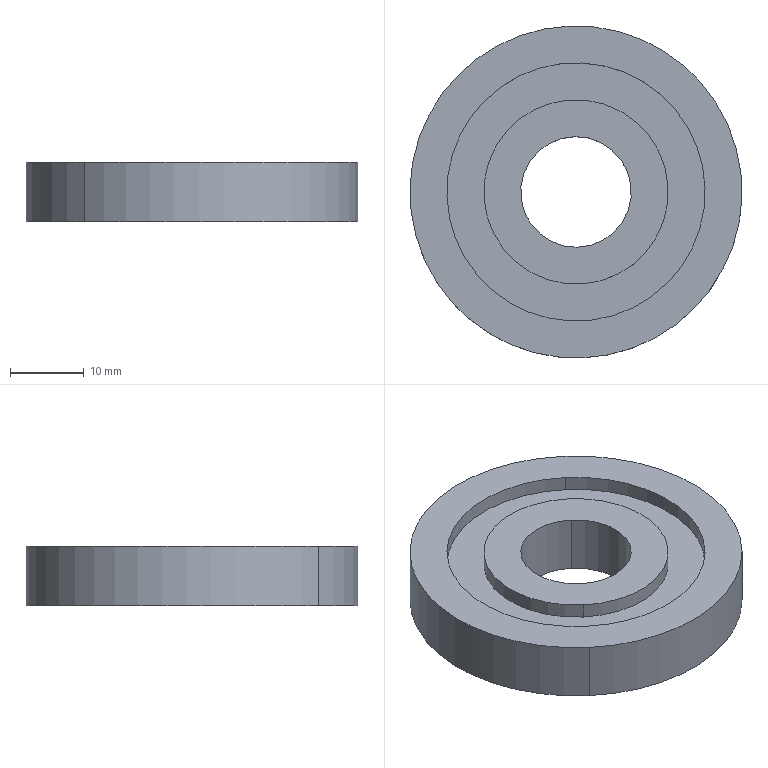Component | SolidWorks | ExcessDoughCuttingWheelBearing-3 | 1 solid | 18 faces | box 45 x 45 x 8 mm | volume 9425 mm3 | cylinder 12 | plane 6 | commonest cylinder face diameters 25 x4 35 x4 15 x2 45 x2
STEP:
#1=CARTESIAN_POINT('',(9.886,-13.898,62.312));
#2=VERTEX_POINT('',#1);
#3=CARTESIAN_POINT('',(9.503,-14.347,62.312));
#4=VERTEX_POINT('',#3);
#5=CARTESIAN_POINT('',(9.695,-14.123,62.312));
#6=DIRECTION('',(0.,0.,1.));
#7=DIRECTION('',(-0.6489,-0.7608,0.));
#8=AXIS2_PLACEMENT_3D('',#5,#6,#7);
#9=CIRCLE('',#8,0.2953);
#10=EDGE_CURVE('',#2,#4,#9,.T.);
#11=ORIENTED_EDGE('',*,*,#10,.F.);
#12=CARTESIAN_POINT('',(9.886,-13.898,62.627));
#13=VERTEX_POINT('',#12);
#14=CARTESIAN_POINT('',(9.886,-13.898,62.684));
#15=DIRECTION('',(0.,0.,1.));
#16=VECTOR('',#15,39.37);
#17=LINE('',#14,#16);
#18=EDGE_CURVE('',#2,#13,#17,.T.);
#19=ORIENTED_EDGE('',*,*,#18,.T.);
#20=CARTESIAN_POINT('',(9.503,-14.347,62.627));
#21=VERTEX_POINT('',#20);
#22=CARTESIAN_POINT('',(9.695,-14.123,62.627));
#23=DIRECTION('',(0.,0.,1.));
#24=DIRECTION('',(-0.6489,-0.7608,0.));
#25=AXIS2_PLACEMENT_3D('',#22,#23,#24);
#26=CIRCLE('',#25,0.2953);
#27=EDGE_CURVE('',#13,#21,#26,.T.);
#28=ORIENTED_EDGE('',*,*,#27,.T.);
#29=CARTESIAN_POINT('',(9.503,-14.347,62.684));
#30=DIRECTION('',(0.,0.,1.));
#31=VECTOR('',#30,39.37);
#32=LINE('',#29,#31);
#33=EDGE_CURVE('',#4,#21,#32,.T.);
#34=ORIENTED_EDGE('',*,*,#33,.F.);
#35=EDGE_LOOP('',(#11,#19,#28,#34));
#36=FACE_OUTER_BOUND('',#35,.T.);
#37=CARTESIAN_POINT('',(9.695,-14.123,62.684));
#38=DIRECTION('',(0.,0.,1.));
#39=DIRECTION('',(-0.6489,-0.7608,0.));
#40=AXIS2_PLACEMENT_3D('',#37,#38,#39);
#41=CYLINDRICAL_SURFACE('',#40,0.2953);
#42=ADVANCED_FACE('',(#36),#41,.F.);
#43=CARTESIAN_POINT('',(9.375,-14.497,62.312));
#44=VERTEX_POINT('',#43);
#45=CARTESIAN_POINT('',(10.014,-13.748,62.312));
#46=VERTEX_POINT('',#45);
#47=CARTESIAN_POINT('',(9.695,-14.123,62.312));
#48=DIRECTION('',(0.,0.,1.));
#49=DIRECTION('',(-0.6489,-0.7608,0.));
#50=AXIS2_PLACEMENT_3D('',#47,#48,#49);
#51=CIRCLE('',#50,0.4921);
#52=EDGE_CURVE('',#44,#46,#51,.T.);
#53=ORIENTED_EDGE('',*,*,#52,.T.);
#54=CARTESIAN_POINT('',(10.014,-13.748,62.391));
#55=VERTEX_POINT('',#54);
#56=CARTESIAN_POINT('',(10.014,-13.748,62.684));
#57=DIRECTION('',(0.,0.,1.));
#58=VECTOR('',#57,39.37);
#59=LINE('',#56,#58);
#60=EDGE_CURVE('',#46,#55,#59,.T.);
#61=ORIENTED_EDGE('',*,*,#60,.T.);
#62=CARTESIAN_POINT('',(9.375,-14.497,62.391));
#63=VERTEX_POINT('',#62);
#64=CARTESIAN_POINT('',(9.695,-14.123,62.391));
#65=DIRECTION('',(0.,0.,1.));
#66=DIRECTION('',(-0.6489,-0.7608,0.));
#67=AXIS2_PLACEMENT_3D('',#64,#65,#66);
#68=CIRCLE('',#67,0.4921);
#69=EDGE_CURVE('',#63,#55,#68,.T.);
#70=ORIENTED_EDGE('',*,*,#69,.F.);
#71=CARTESIAN_POINT('',(9.375,-14.497,62.684));
#72=DIRECTION('',(0.,0.,1.));
#73=VECTOR('',#72,39.37);
#74=LINE('',#71,#73);
#75=EDGE_CURVE('',#44,#63,#74,.T.);
#76=ORIENTED_EDGE('',*,*,#75,.F.);
#77=EDGE_LOOP('',(#53,#61,#70,#76));
#78=FACE_OUTER_BOUND('',#77,.T.);
#79=CARTESIAN_POINT('',(9.695,-14.123,62.684));
#80=DIRECTION('',(0.,0.,1.));
#81=DIRECTION('',(-0.6489,-0.7608,0.));
#82=AXIS2_PLACEMENT_3D('',#79,#80,#81);
#83=CYLINDRICAL_SURFACE('',#82,0.4921);
#84=ADVANCED_FACE('',(#78),#83,.T.);
#85=CARTESIAN_POINT('',(10.142,-13.598,62.312));
#86=VERTEX_POINT('',#85);
#87=CARTESIAN_POINT('',(9.247,-14.647,62.312));
#88=VERTEX_POINT('',#87);
#89=CARTESIAN_POINT('',(9.695,-14.123,62.312));
#90=DIRECTION('',(0.,0.,1.));
#91=DIRECTION('',(-0.6489,-0.7608,0.));
#92=AXIS2_PLACEMENT_3D('',#89,#90,#91);
#93=CIRCLE('',#92,0.689);
#94=EDGE_CURVE('',#86,#88,#93,.T.);
#95=ORIENTED_EDGE('',*,*,#94,.F.);
#96=CARTESIAN_POINT('',(10.142,-13.598,62.391));
#97=VERTEX_POINT('',#96);
#98=CARTESIAN_POINT('',(10.142,-13.598,62.684));
#99=DIRECTION('',(0.,0.,1.));
#100=VECTOR('',#99,39.37);
#101=LINE('',#98,#100);
#102=EDGE_CURVE('',#86,#97,#101,.T.);
#103=ORIENTED_EDGE('',*,*,#102,.T.);
#104=CARTESIAN_POINT('',(9.247,-14.647,62.391));
#105=VERTEX_POINT('',#104);
#106=CARTESIAN_POINT('',(9.695,-14.123,62.391));
#107=DIRECTION('',(0.,0.,1.));
#108=DIRECTION('',(-0.6489,-0.7608,0.));
#109=AXIS2_PLACEMENT_3D('',#106,#107,#108);
#110=CIRCLE('',#109,0.689);
#111=EDGE_CURVE('',#97,#105,#110,.T.);
#112=ORIENTED_EDGE('',*,*,#111,.T.);
#113=CARTESIAN_POINT('',(9.247,-14.647,62.684));
#114=DIRECTION('',(0.,0.,1.));
#115=VECTOR('',#114,39.37);
#116=LINE('',#113,#115);
#117=EDGE_CURVE('',#88,#105,#116,.T.);
#118=ORIENTED_EDGE('',*,*,#117,.F.);
#119=EDGE_LOOP('',(#95,#103,#112,#118));
#120=FACE_OUTER_BOUND('',#119,.T.);
#121=CARTESIAN_POINT('',(9.695,-14.123,62.684));
#122=DIRECTION('',(0.,0.,1.));
#123=DIRECTION('',(-0.6489,-0.7608,0.));
#124=AXIS2_PLACEMENT_3D('',#121,#122,#123);
#125=CYLINDRICAL_SURFACE('',#124,0.689);
#126=ADVANCED_FACE('',(#120),#125,.F.);
#127=CARTESIAN_POINT('',(9.12,-14.797,62.312));
#128=VERTEX_POINT('',#127);
#129=CARTESIAN_POINT('',(10.269,-13.449,62.312));
#130=VERTEX_POINT('',#129);
#131=CARTESIAN_POINT('',(9.695,-14.123,62.312));
#132=DIRECTION('',(0.,0.,1.));
#133=DIRECTION('',(-0.6489,-0.7608,0.));
#134=AXIS2_PLACEMENT_3D('',#131,#132,#133);
#135=CIRCLE('',#134,0.8858);
#136=EDGE_CURVE('',#128,#130,#135,.T.);
#137=ORIENTED_EDGE('',*,*,#136,.T.);
#138=CARTESIAN_POINT('',(10.269,-13.449,62.627));
#139=VERTEX_POINT('',#138);
#140=CARTESIAN_POINT('',(10.269,-13.449,62.684));
#141=DIRECTION('',(0.,0.,1.));
#142=VECTOR('',#141,39.37);
#143=LINE('',#140,#142);
#144=EDGE_CURVE('',#130,#139,#143,.T.);
#145=ORIENTED_EDGE('',*,*,#144,.T.);
#146=CARTESIAN_POINT('',(9.12,-14.797,62.627));
#147=VERTEX_POINT('',#146);
#148=CARTESIAN_POINT('',(9.695,-14.123,62.627));
#149=DIRECTION('',(0.,0.,1.));
#150=DIRECTION('',(-0.6489,-0.7608,0.));
#151=AXIS2_PLACEMENT_3D('',#148,#149,#150);
#152=CIRCLE('',#151,0.8858);
#153=EDGE_CURVE('',#147,#139,#152,.T.);
#154=ORIENTED_EDGE('',*,*,#153,.F.);
#155=CARTESIAN_POINT('',(9.12,-14.797,62.684));
#156=DIRECTION('',(0.,0.,1.));
#157=VECTOR('',#156,39.37);
#158=LINE('',#155,#157);
#159=EDGE_CURVE('',#128,#147,#158,.T.);
#160=ORIENTED_EDGE('',*,*,#159,.F.);
#161=EDGE_LOOP('',(#137,#145,#154,#160));
#162=FACE_OUTER_BOUND('',#161,.T.);
#163=CARTESIAN_POINT('',(9.695,-14.123,62.684));
#164=DIRECTION('',(0.,0.,1.));
#165=DIRECTION('',(-0.6489,-0.7608,0.));
#166=AXIS2_PLACEMENT_3D('',#163,#164,#165);
#167=CYLINDRICAL_SURFACE('',#166,0.8858);
#168=ADVANCED_FACE('',(#162),#167,.T.);
#169=CARTESIAN_POINT('',(10.142,-13.598,62.548));
#170=VERTEX_POINT('',#169);
#171=CARTESIAN_POINT('',(9.247,-14.647,62.548));
#172=VERTEX_POINT('',#171);
#173=CARTESIAN_POINT('',(9.695,-14.123,62.548));
#174=DIRECTION('',(0.,0.,1.));
#175=DIRECTION('',(-0.6489,-0.7608,0.));
#176=AXIS2_PLACEMENT_3D('',#173,#174,#175);
#177=CIRCLE('',#176,0.689);
#178=EDGE_CURVE('',#170,#172,#177,.T.);
#179=ORIENTED_EDGE('',*,*,#178,.F.);
#180=CARTESIAN_POINT('',(10.142,-13.598,62.627));
#181=VERTEX_POINT('',#180);
#182=CARTESIAN_POINT('',(10.142,-13.598,62.684));
#183=DIRECTION('',(0.,0.,1.));
#184=VECTOR('',#183,39.37);
#185=LINE('',#182,#184);
#186=EDGE_CURVE('',#170,#181,#185,.T.);
#187=ORIENTED_EDGE('',*,*,#186,.T.);
#188=CARTESIAN_POINT('',(9.247,-14.647,62.627));
#189=VERTEX_POINT('',#188);
#190=CARTESIAN_POINT('',(9.695,-14.123,62.627));
#191=DIRECTION('',(0.,0.,1.));
#192=DIRECTION('',(-0.6489,-0.7608,0.));
#193=AXIS2_PLACEMENT_3D('',#190,#191,#192);
#194=CIRCLE('',#193,0.689);
#195=EDGE_CURVE('',#181,#189,#194,.T.);
#196=ORIENTED_EDGE('',*,*,#195,.T.);
#197=CARTESIAN_POINT('',(9.247,-14.647,62.684));
#198=DIRECTION('',(0.,0.,1.));
#199=VECTOR('',#198,39.37);
#200=LINE('',#197,#199);
#201=EDGE_CURVE('',#172,#189,#200,.T.);
#202=ORIENTED_EDGE('',*,*,#201,.F.);
#203=EDGE_LOOP('',(#179,#187,#196,#202));
#204=FACE_OUTER_BOUND('',#203,.T.);
#205=CARTESIAN_POINT('',(9.695,-14.123,62.684));
#206=DIRECTION('',(0.,0.,1.));
#207=DIRECTION('',(-0.6489,-0.7608,0.));
#208=AXIS2_PLACEMENT_3D('',#205,#206,#207);
#209=CYLINDRICAL_SURFACE('',#208,0.689);
#210=ADVANCED_FACE('',(#204),#209,.F.);
#211=CARTESIAN_POINT('',(9.375,-14.497,62.548));
#212=VERTEX_POINT('',#211);
#213=CARTESIAN_POINT('',(10.014,-13.748,62.548));
#214=VERTEX_POINT('',#213);
#215=CARTESIAN_POINT('',(9.695,-14.123,62.548));
#216=DIRECTION('',(0.,0.,1.));
#217=DIRECTION('',(-0.6489,-0.7608,0.));
#218=AXIS2_PLACEMENT_3D('',#215,#216,#217);
#219=CIRCLE('',#218,0.4921);
#220=EDGE_CURVE('',#212,#214,#219,.T.);
#221=ORIENTED_EDGE('',*,*,#220,.T.);
#222=CARTESIAN_POINT('',(10.014,-13.748,62.627));
#223=VERTEX_POINT('',#222);
#224=CARTESIAN_POINT('',(10.014,-13.748,62.684));
#225=DIRECTION('',(0.,0.,1.));
#226=VECTOR('',#225,39.37);
#227=LINE('',#224,#226);
#228=EDGE_CURVE('',#214,#223,#227,.T.);
#229=ORIENTED_EDGE('',*,*,#228,.T.);
#230=CARTESIAN_POINT('',(9.375,-14.497,62.627));
#231=VERTEX_POINT('',#230);
#232=CARTESIAN_POINT('',(9.695,-14.123,62.627));
#233=DIRECTION('',(0.,0.,1.));
#234=DIRECTION('',(-0.6489,-0.7608,0.));
#235=AXIS2_PLACEMENT_3D('',#232,#233,#234);
#236=CIRCLE('',#235,0.4921);
#237=EDGE_CURVE('',#231,#223,#236,.T.);
#238=ORIENTED_EDGE('',*,*,#237,.F.);
#239=CARTESIAN_POINT('',(9.375,-14.497,62.684));
#240=DIRECTION('',(0.,0.,1.));
#241=VECTOR('',#240,39.37);
#242=LINE('',#239,#241);
#243=EDGE_CURVE('',#212,#231,#242,.T.);
#244=ORIENTED_EDGE('',*,*,#243,.F.);
#245=EDGE_LOOP('',(#221,#229,#238,#244));
#246=FACE_OUTER_BOUND('',#245,.T.);
#247=CARTESIAN_POINT('',(9.695,-14.123,62.684));
#248=DIRECTION('',(0.,0.,1.));
#249=DIRECTION('',(-0.6489,-0.7608,0.));
#250=AXIS2_PLACEMENT_3D('',#247,#248,#249);
#251=CYLINDRICAL_SURFACE('',#250,0.4921);
#252=ADVANCED_FACE('',(#246),#251,.T.);
#253=CARTESIAN_POINT('',(9.695,-14.123,62.627));
#254=DIRECTION('',(0.,0.,1.));
#255=DIRECTION('',(-0.6489,-0.7608,0.));
#256=AXIS2_PLACEMENT_3D('',#253,#254,#255);
#257=CIRCLE('',#256,0.2953);
#258=EDGE_CURVE('',#21,#13,#257,.T.);
#259=ORIENTED_EDGE('',*,*,#258,.F.);
#260=ORIENTED_EDGE('',*,*,#27,.F.);
#261=EDGE_LOOP('',(#259,#260));
#262=FACE_BOUND('',#261,.T.);
#263=ORIENTED_EDGE('',*,*,#237,.T.);
#264=CARTESIAN_POINT('',(9.695,-14.123,62.627));
#265=DIRECTION('',(0.,0.,1.));
#266=DIRECTION('',(-0.6489,-0.7608,0.));
#267=AXIS2_PLACEMENT_3D('',#264,#265,#266);
#268=CIRCLE('',#267,0.4921);
#269=EDGE_CURVE('',#223,#231,#268,.T.);
#270=ORIENTED_EDGE('',*,*,#269,.T.);
#271=EDGE_LOOP('',(#263,#270));
#272=FACE_OUTER_BOUND('',#271,.T.);
#273=CARTESIAN_POINT('',(9.886,-13.898,62.627));
#274=DIRECTION('',(0.,0.,-1.));
#275=DIRECTION('',(0.6489,0.7608,0.));
#276=AXIS2_PLACEMENT_3D('',#273,#274,#275);
#277=PLANE('',#276);
#278=ADVANCED_FACE('',(#262,#272),#277,.F.);
#279=ORIENTED_EDGE('',*,*,#228,.F.);
#280=CARTESIAN_POINT('',(9.695,-14.123,62.548));
#281=DIRECTION('',(0.,0.,1.));
#282=DIRECTION('',(-0.6489,-0.7608,0.));
#283=AXIS2_PLACEMENT_3D('',#280,#281,#282);
#284=CIRCLE('',#283,0.4921);
#285=EDGE_CURVE('',#214,#212,#284,.T.);
#286=ORIENTED_EDGE('',*,*,#285,.T.);
#287=ORIENTED_EDGE('',*,*,#243,.T.);
#288=ORIENTED_EDGE('',*,*,#269,.F.);
#289=EDGE_LOOP('',(#279,#286,#287,#288));
#290=FACE_OUTER_BOUND('',#289,.T.);
#291=CARTESIAN_POINT('',(9.695,-14.123,62.684));
#292=DIRECTION('',(0.,0.,1.));
#293=DIRECTION('',(-0.6489,-0.7608,0.));
#294=AXIS2_PLACEMENT_3D('',#291,#292,#293);
#295=CYLINDRICAL_SURFACE('',#294,0.4921);
#296=ADVANCED_FACE('',(#290),#295,.T.);
#297=ORIENTED_EDGE('',*,*,#220,.F.);
#298=ORIENTED_EDGE('',*,*,#285,.F.);
#299=EDGE_LOOP('',(#297,#298));
#300=FACE_BOUND('',#299,.T.);
#301=CARTESIAN_POINT('',(9.695,-14.123,62.548));
#302=DIRECTION('',(0.,0.,1.));
#303=DIRECTION('',(-0.6489,-0.7608,0.));
#304=AXIS2_PLACEMENT_3D('',#301,#302,#303);
#305=CIRCLE('',#304,0.689);
#306=EDGE_CURVE('',#172,#170,#305,.T.);
#307=ORIENTED_EDGE('',*,*,#306,.T.);
#308=ORIENTED_EDGE('',*,*,#178,.T.);
#309=EDGE_LOOP('',(#307,#308));
#310=FACE_OUTER_BOUND('',#309,.T.);
#311=CARTESIAN_POINT('',(10.014,-13.748,62.548));
#312=DIRECTION('',(0.,0.,-1.));
#313=DIRECTION('',(0.6489,0.7608,0.));
#314=AXIS2_PLACEMENT_3D('',#311,#312,#313);
#315=PLANE('',#314);
#316=ADVANCED_FACE('',(#300,#310),#315,.F.);
#317=ORIENTED_EDGE('',*,*,#186,.F.);
#318=ORIENTED_EDGE('',*,*,#306,.F.);
#319=ORIENTED_EDGE('',*,*,#201,.T.);
#320=CARTESIAN_POINT('',(9.695,-14.123,62.627));
#321=DIRECTION('',(0.,0.,1.));
#322=DIRECTION('',(-0.6489,-0.7608,0.));
#323=AXIS2_PLACEMENT_3D('',#320,#321,#322);
#324=CIRCLE('',#323,0.689);
#325=EDGE_CURVE('',#189,#181,#324,.T.);
#326=ORIENTED_EDGE('',*,*,#325,.T.);
#327=EDGE_LOOP('',(#317,#318,#319,#326));
#328=FACE_OUTER_BOUND('',#327,.T.);
#329=CARTESIAN_POINT('',(9.695,-14.123,62.684));
#330=DIRECTION('',(0.,0.,1.));
#331=DIRECTION('',(-0.6489,-0.7608,0.));
#332=AXIS2_PLACEMENT_3D('',#329,#330,#331);
#333=CYLINDRICAL_SURFACE('',#332,0.689);
#334=ADVANCED_FACE('',(#328),#333,.F.);
#335=ORIENTED_EDGE('',*,*,#325,.F.);
#336=ORIENTED_EDGE('',*,*,#195,.F.);
#337=EDGE_LOOP('',(#335,#336));
#338=FACE_BOUND('',#337,.T.);
#339=ORIENTED_EDGE('',*,*,#153,.T.);
#340=CARTESIAN_POINT('',(9.695,-14.123,62.627));
#341=DIRECTION('',(0.,0.,1.));
#342=DIRECTION('',(-0.6489,-0.7608,0.));
#343=AXIS2_PLACEMENT_3D('',#340,#341,#342);
#344=CIRCLE('',#343,0.8858);
#345=EDGE_CURVE('',#139,#147,#344,.T.);
#346=ORIENTED_EDGE('',*,*,#345,.T.);
#347=EDGE_LOOP('',(#339,#346));
#348=FACE_OUTER_BOUND('',#347,.T.);
#349=CARTESIAN_POINT('',(10.142,-13.598,62.627));
#350=DIRECTION('',(0.,0.,-1.));
#351=DIRECTION('',(0.6489,0.7608,0.));
#352=AXIS2_PLACEMENT_3D('',#349,#350,#351);
#353=PLANE('',#352);
#354=ADVANCED_FACE('',(#338,#348),#353,.F.);
#355=ORIENTED_EDGE('',*,*,#144,.F.);
#356=CARTESIAN_POINT('',(9.695,-14.123,62.312));
#357=DIRECTION('',(0.,0.,1.));
#358=DIRECTION('',(-0.6489,-0.7608,0.));
#359=AXIS2_PLACEMENT_3D('',#356,#357,#358);
#360=CIRCLE('',#359,0.8858);
#361=EDGE_CURVE('',#130,#128,#360,.T.);
#362=ORIENTED_EDGE('',*,*,#361,.T.);
#363=ORIENTED_EDGE('',*,*,#159,.T.);
#364=ORIENTED_EDGE('',*,*,#345,.F.);
#365=EDGE_LOOP('',(#355,#362,#363,#364));
#366=FACE_OUTER_BOUND('',#365,.T.);
#367=CARTESIAN_POINT('',(9.695,-14.123,62.684));
#368=DIRECTION('',(0.,0.,1.));
#369=DIRECTION('',(-0.6489,-0.7608,0.));
#370=AXIS2_PLACEMENT_3D('',#367,#368,#369);
#371=CYLINDRICAL_SURFACE('',#370,0.8858);
#372=ADVANCED_FACE('',(#366),#371,.T.);
#373=ORIENTED_EDGE('',*,*,#136,.F.);
#374=ORIENTED_EDGE('',*,*,#361,.F.);
#375=EDGE_LOOP('',(#373,#374));
#376=FACE_OUTER_BOUND('',#375,.T.);
#377=CARTESIAN_POINT('',(9.695,-14.123,62.312));
#378=DIRECTION('',(0.,0.,1.));
#379=DIRECTION('',(-0.6489,-0.7608,0.));
#380=AXIS2_PLACEMENT_3D('',#377,#378,#379);
#381=CIRCLE('',#380,0.689);
#382=EDGE_CURVE('',#88,#86,#381,.T.);
#383=ORIENTED_EDGE('',*,*,#382,.T.);
#384=ORIENTED_EDGE('',*,*,#94,.T.);
#385=EDGE_LOOP('',(#383,#384));
#386=FACE_BOUND('',#385,.T.);
#387=CARTESIAN_POINT('',(10.269,-13.449,62.312));
#388=DIRECTION('',(0.,0.,1.));
#389=DIRECTION('',(-0.6489,-0.7608,0.));
#390=AXIS2_PLACEMENT_3D('',#387,#388,#389);
#391=PLANE('',#390);
#392=ADVANCED_FACE('',(#376,#386),#391,.F.);
#393=ORIENTED_EDGE('',*,*,#102,.F.);
#394=ORIENTED_EDGE('',*,*,#382,.F.);
#395=ORIENTED_EDGE('',*,*,#117,.T.);
#396=CARTESIAN_POINT('',(9.695,-14.123,62.391));
#397=DIRECTION('',(0.,0.,1.));
#398=DIRECTION('',(-0.6489,-0.7608,0.));
#399=AXIS2_PLACEMENT_3D('',#396,#397,#398);
#400=CIRCLE('',#399,0.689);
#401=EDGE_CURVE('',#105,#97,#400,.T.);
#402=ORIENTED_EDGE('',*,*,#401,.T.);
#403=EDGE_LOOP('',(#393,#394,#395,#402));
#404=FACE_OUTER_BOUND('',#403,.T.);
#405=CARTESIAN_POINT('',(9.695,-14.123,62.684));
#406=DIRECTION('',(0.,0.,1.));
#407=DIRECTION('',(-0.6489,-0.7608,0.));
#408=AXIS2_PLACEMENT_3D('',#405,#406,#407);
#409=CYLINDRICAL_SURFACE('',#408,0.689);
#410=ADVANCED_FACE('',(#404),#409,.F.);
#411=ORIENTED_EDGE('',*,*,#401,.F.);
#412=ORIENTED_EDGE('',*,*,#111,.F.);
#413=EDGE_LOOP('',(#411,#412));
#414=FACE_OUTER_BOUND('',#413,.T.);
#415=ORIENTED_EDGE('',*,*,#69,.T.);
#416=CARTESIAN_POINT('',(9.695,-14.123,62.391));
#417=DIRECTION('',(0.,0.,1.));
#418=DIRECTION('',(-0.6489,-0.7608,0.));
#419=AXIS2_PLACEMENT_3D('',#416,#417,#418);
#420=CIRCLE('',#419,0.4921);
#421=EDGE_CURVE('',#55,#63,#420,.T.);
#422=ORIENTED_EDGE('',*,*,#421,.T.);
#423=EDGE_LOOP('',(#415,#422));
#424=FACE_BOUND('',#423,.T.);
#425=CARTESIAN_POINT('',(10.142,-13.598,62.391));
#426=DIRECTION('',(0.,0.,1.));
#427=DIRECTION('',(-0.6489,-0.7608,0.));
#428=AXIS2_PLACEMENT_3D('',#425,#426,#427);
#429=PLANE('',#428);
#430=ADVANCED_FACE('',(#414,#424),#429,.F.);
#431=ORIENTED_EDGE('',*,*,#60,.F.);
#432=CARTESIAN_POINT('',(9.695,-14.123,62.312));
#433=DIRECTION('',(0.,0.,1.));
#434=DIRECTION('',(-0.6489,-0.7608,0.));
#435=AXIS2_PLACEMENT_3D('',#432,#433,#434);
#436=CIRCLE('',#435,0.4921);
#437=EDGE_CURVE('',#46,#44,#436,.T.);
#438=ORIENTED_EDGE('',*,*,#437,.T.);
#439=ORIENTED_EDGE('',*,*,#75,.T.);
#440=ORIENTED_EDGE('',*,*,#421,.F.);
#441=EDGE_LOOP('',(#431,#438,#439,#440));
#442=FACE_OUTER_BOUND('',#441,.T.);
#443=CARTESIAN_POINT('',(9.695,-14.123,62.684));
#444=DIRECTION('',(0.,0.,1.));
#445=DIRECTION('',(-0.6489,-0.7608,0.));
#446=AXIS2_PLACEMENT_3D('',#443,#444,#445);
#447=CYLINDRICAL_SURFACE('',#446,0.4921);
#448=ADVANCED_FACE('',(#442),#447,.T.);
#449=ORIENTED_EDGE('',*,*,#52,.F.);
#450=ORIENTED_EDGE('',*,*,#437,.F.);
#451=EDGE_LOOP('',(#449,#450));
#452=FACE_OUTER_BOUND('',#451,.T.);
#453=CARTESIAN_POINT('',(9.695,-14.123,62.312));
#454=DIRECTION('',(0.,0.,1.));
#455=DIRECTION('',(-0.6489,-0.7608,0.));
#456=AXIS2_PLACEMENT_3D('',#453,#454,#455);
#457=CIRCLE('',#456,0.2953);
#458=EDGE_CURVE('',#4,#2,#457,.T.);
#459=ORIENTED_EDGE('',*,*,#458,.T.);
#460=ORIENTED_EDGE('',*,*,#10,.T.);
#461=EDGE_LOOP('',(#459,#460));
#462=FACE_BOUND('',#461,.T.);
#463=CARTESIAN_POINT('',(10.014,-13.748,62.312));
#464=DIRECTION('',(0.,0.,1.));
#465=DIRECTION('',(-0.6489,-0.7608,0.));
#466=AXIS2_PLACEMENT_3D('',#463,#464,#465);
#467=PLANE('',#466);
#468=ADVANCED_FACE('',(#452,#462),#467,.F.);
#469=ORIENTED_EDGE('',*,*,#18,.F.);
#470=ORIENTED_EDGE('',*,*,#458,.F.);
#471=ORIENTED_EDGE('',*,*,#33,.T.);
#472=ORIENTED_EDGE('',*,*,#258,.T.);
#473=EDGE_LOOP('',(#469,#470,#471,#472));
#474=FACE_OUTER_BOUND('',#473,.T.);
#475=CARTESIAN_POINT('',(9.695,-14.123,62.684));
#476=DIRECTION('',(0.,0.,1.));
#477=DIRECTION('',(-0.6489,-0.7608,0.));
#478=AXIS2_PLACEMENT_3D('',#475,#476,#477);
#479=CYLINDRICAL_SURFACE('',#478,0.2953);
#480=ADVANCED_FACE('',(#474),#479,.F.);
#481=CLOSED_SHELL('',(#42,#84,#126,#168,#210,#252,#278,#296,#316,#334,#354,#372,#392,#410,#430,#448,#468,#480));
#482=MANIFOLD_SOLID_BREP('',#481);
#483=CARTESIAN_POINT('',(0.,0.,0.));
#484=DIRECTION('',(0.,0.,1.));
#485=DIRECTION('',(1.,0.,0.));
#486=AXIS2_PLACEMENT_3D('',#483,#484,#485);
#487=(LENGTH_UNIT()NAMED_UNIT(*)SI_UNIT($,.METRE.));
#488=LENGTH_MEASURE_WITH_UNIT(LENGTH_MEASURE(0.0254),#487);
#489=DIMENSIONAL_EXPONENTS(1.,0.,0.,0.,0.,0.,0.);
#490=(CONVERSION_BASED_UNIT('',#488)LENGTH_UNIT()NAMED_UNIT(#489));
#491=UNCERTAINTY_MEASURE_WITH_UNIT(LENGTH_MEASURE(0.00001),#490,'','');
#492=(NAMED_UNIT(*)PLANE_ANGLE_UNIT()SI_UNIT($,.RADIAN.));
#493=(NAMED_UNIT(*)SI_UNIT($,.STERADIAN.)SOLID_ANGLE_UNIT());
#494=(GEOMETRIC_REPRESENTATION_CONTEXT(3)GLOBAL_UNCERTAINTY_ASSIGNED_CONTEXT((#491))GLOBAL_UNIT_ASSIGNED_CONTEXT((#490,#492,#493))REPRESENTATION_CONTEXT('',''));
#495=ADVANCED_BREP_SHAPE_REPRESENTATION('',(#482,#486),#494);
#496=COLOUR_RGB('',0.7922,0.8196,0.9333);
#497=FILL_AREA_STYLE_COLOUR('',#496);
#498=FILL_AREA_STYLE('',(#497));
#499=SURFACE_STYLE_FILL_AREA(#498);
#500=SURFACE_SIDE_STYLE('',(#499));
#501=SURFACE_STYLE_USAGE(.BOTH.,#500);
#502=PRESENTATION_STYLE_ASSIGNMENT((#501));
#503=STYLED_ITEM('',(#502),#482);
#504=PRESENTATION_LAYER_ASSIGNMENT('','',(#503));
#505=(LENGTH_UNIT()NAMED_UNIT(*)SI_UNIT($,.METRE.));
#506=LENGTH_MEASURE_WITH_UNIT(LENGTH_MEASURE(0.0254),#505);
#507=DIMENSIONAL_EXPONENTS(1.,0.,0.,0.,0.,0.,0.);
#508=(CONVERSION_BASED_UNIT('',#506)LENGTH_UNIT()NAMED_UNIT(#507));
#509=UNCERTAINTY_MEASURE_WITH_UNIT(LENGTH_MEASURE(0.00001),#508,'','');
#510=(NAMED_UNIT(*)PLANE_ANGLE_UNIT()SI_UNIT($,.RADIAN.));
#511=(NAMED_UNIT(*)SI_UNIT($,.STERADIAN.)SOLID_ANGLE_UNIT());
#512=(GEOMETRIC_REPRESENTATION_CONTEXT(3)GLOBAL_UNCERTAINTY_ASSIGNED_CONTEXT((#509))GLOBAL_UNIT_ASSIGNED_CONTEXT((#508,#510,#511))REPRESENTATION_CONTEXT('',''));
#513=MECHANICAL_DESIGN_GEOMETRIC_PRESENTATION_REPRESENTATION('',(#503),#512);